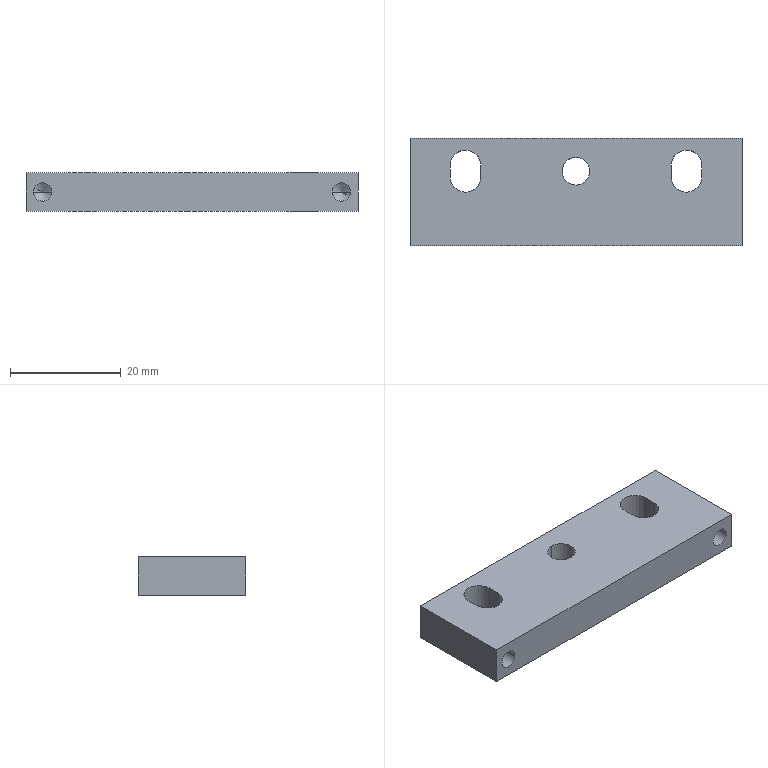CAM job | Mastercam | mm | 10 operations | part box 60 x 19.5 x 7
1. Facing | 24 - 100 平铣刀
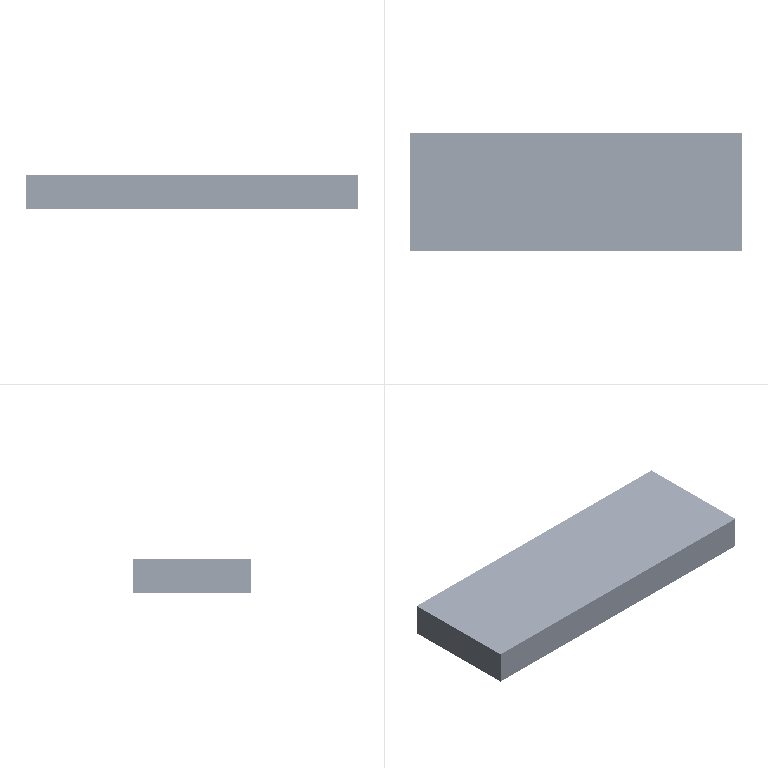2. 2D High Speed (2D Dynamic Mill) | 9 - 10 平铣刀
3. Contour (2D) | 10 - 10 平铣刀
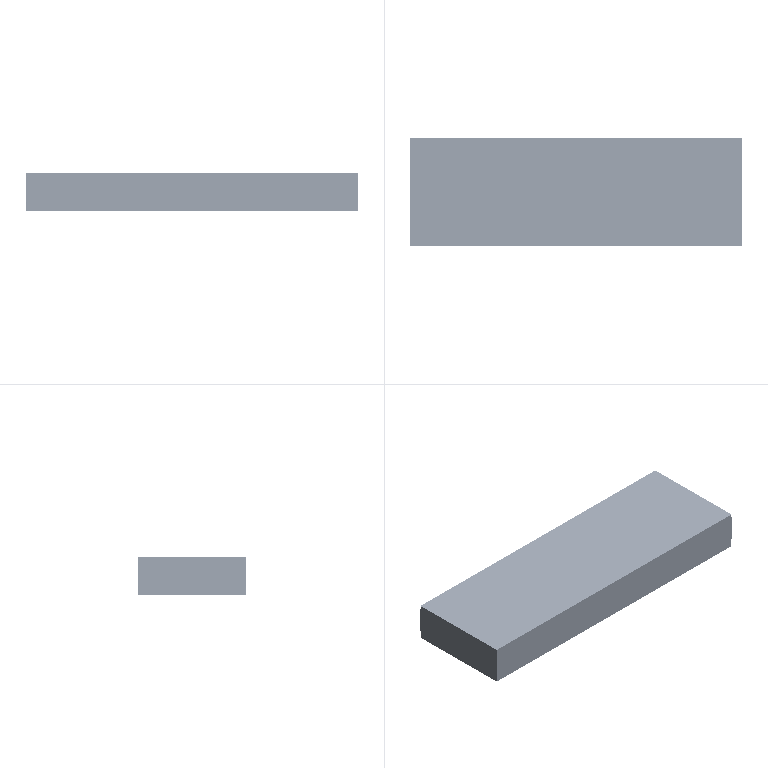4. Contour (Ramp) | 3 - 3 平铣刀
5. Contour (Ramp) | 3 - 3 平铣刀
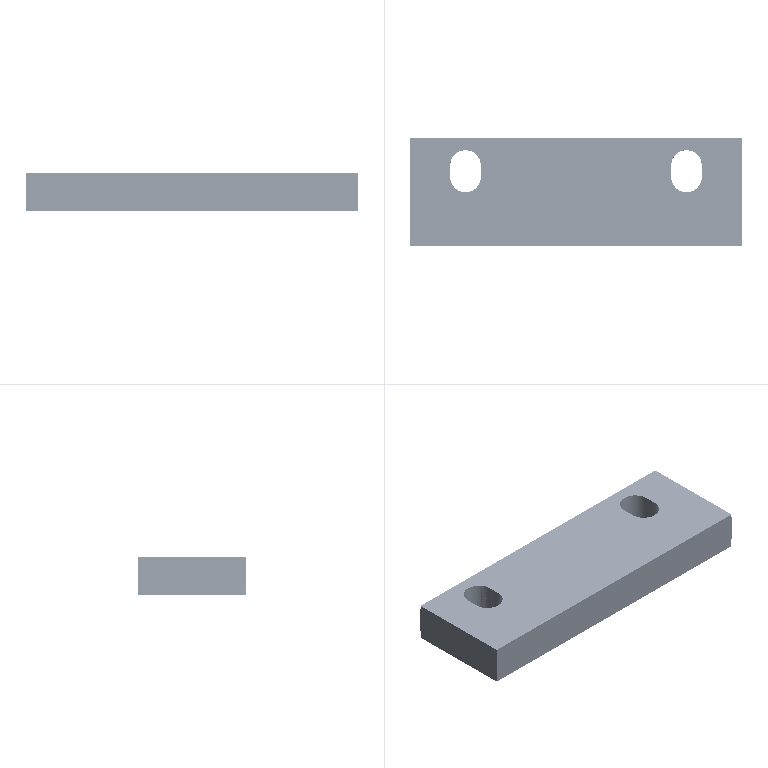6. Drill/Counterbore | 5 - 4 倒角刀
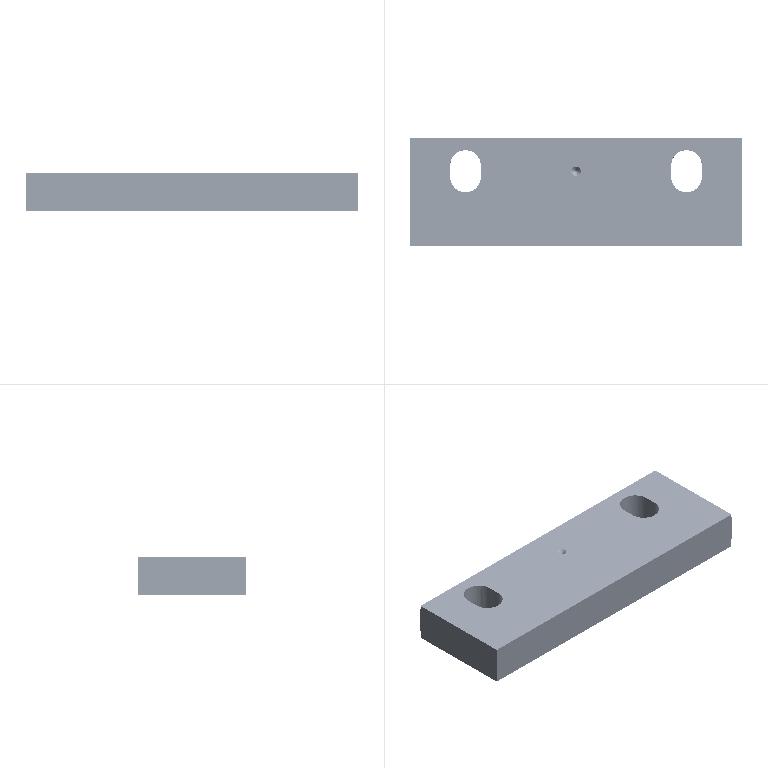7. Contour (2D chamfer) | 5 - 4 倒角刀
8. Facing | 24 - 100 平铣刀
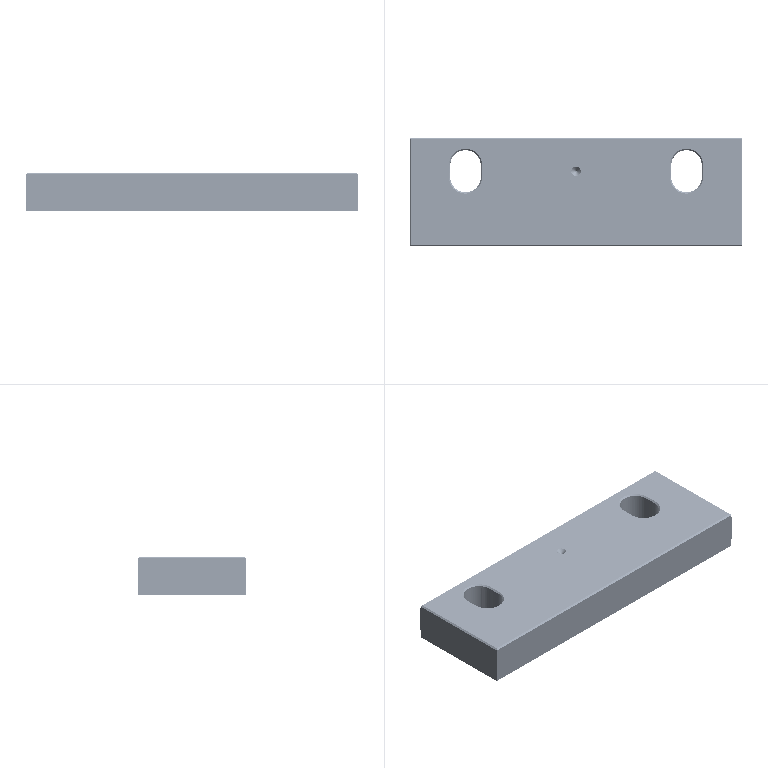9. Contour (2D chamfer) | 5 - 4 倒角刀
10. Drill/Counterbore | 5 - 4 倒角刀